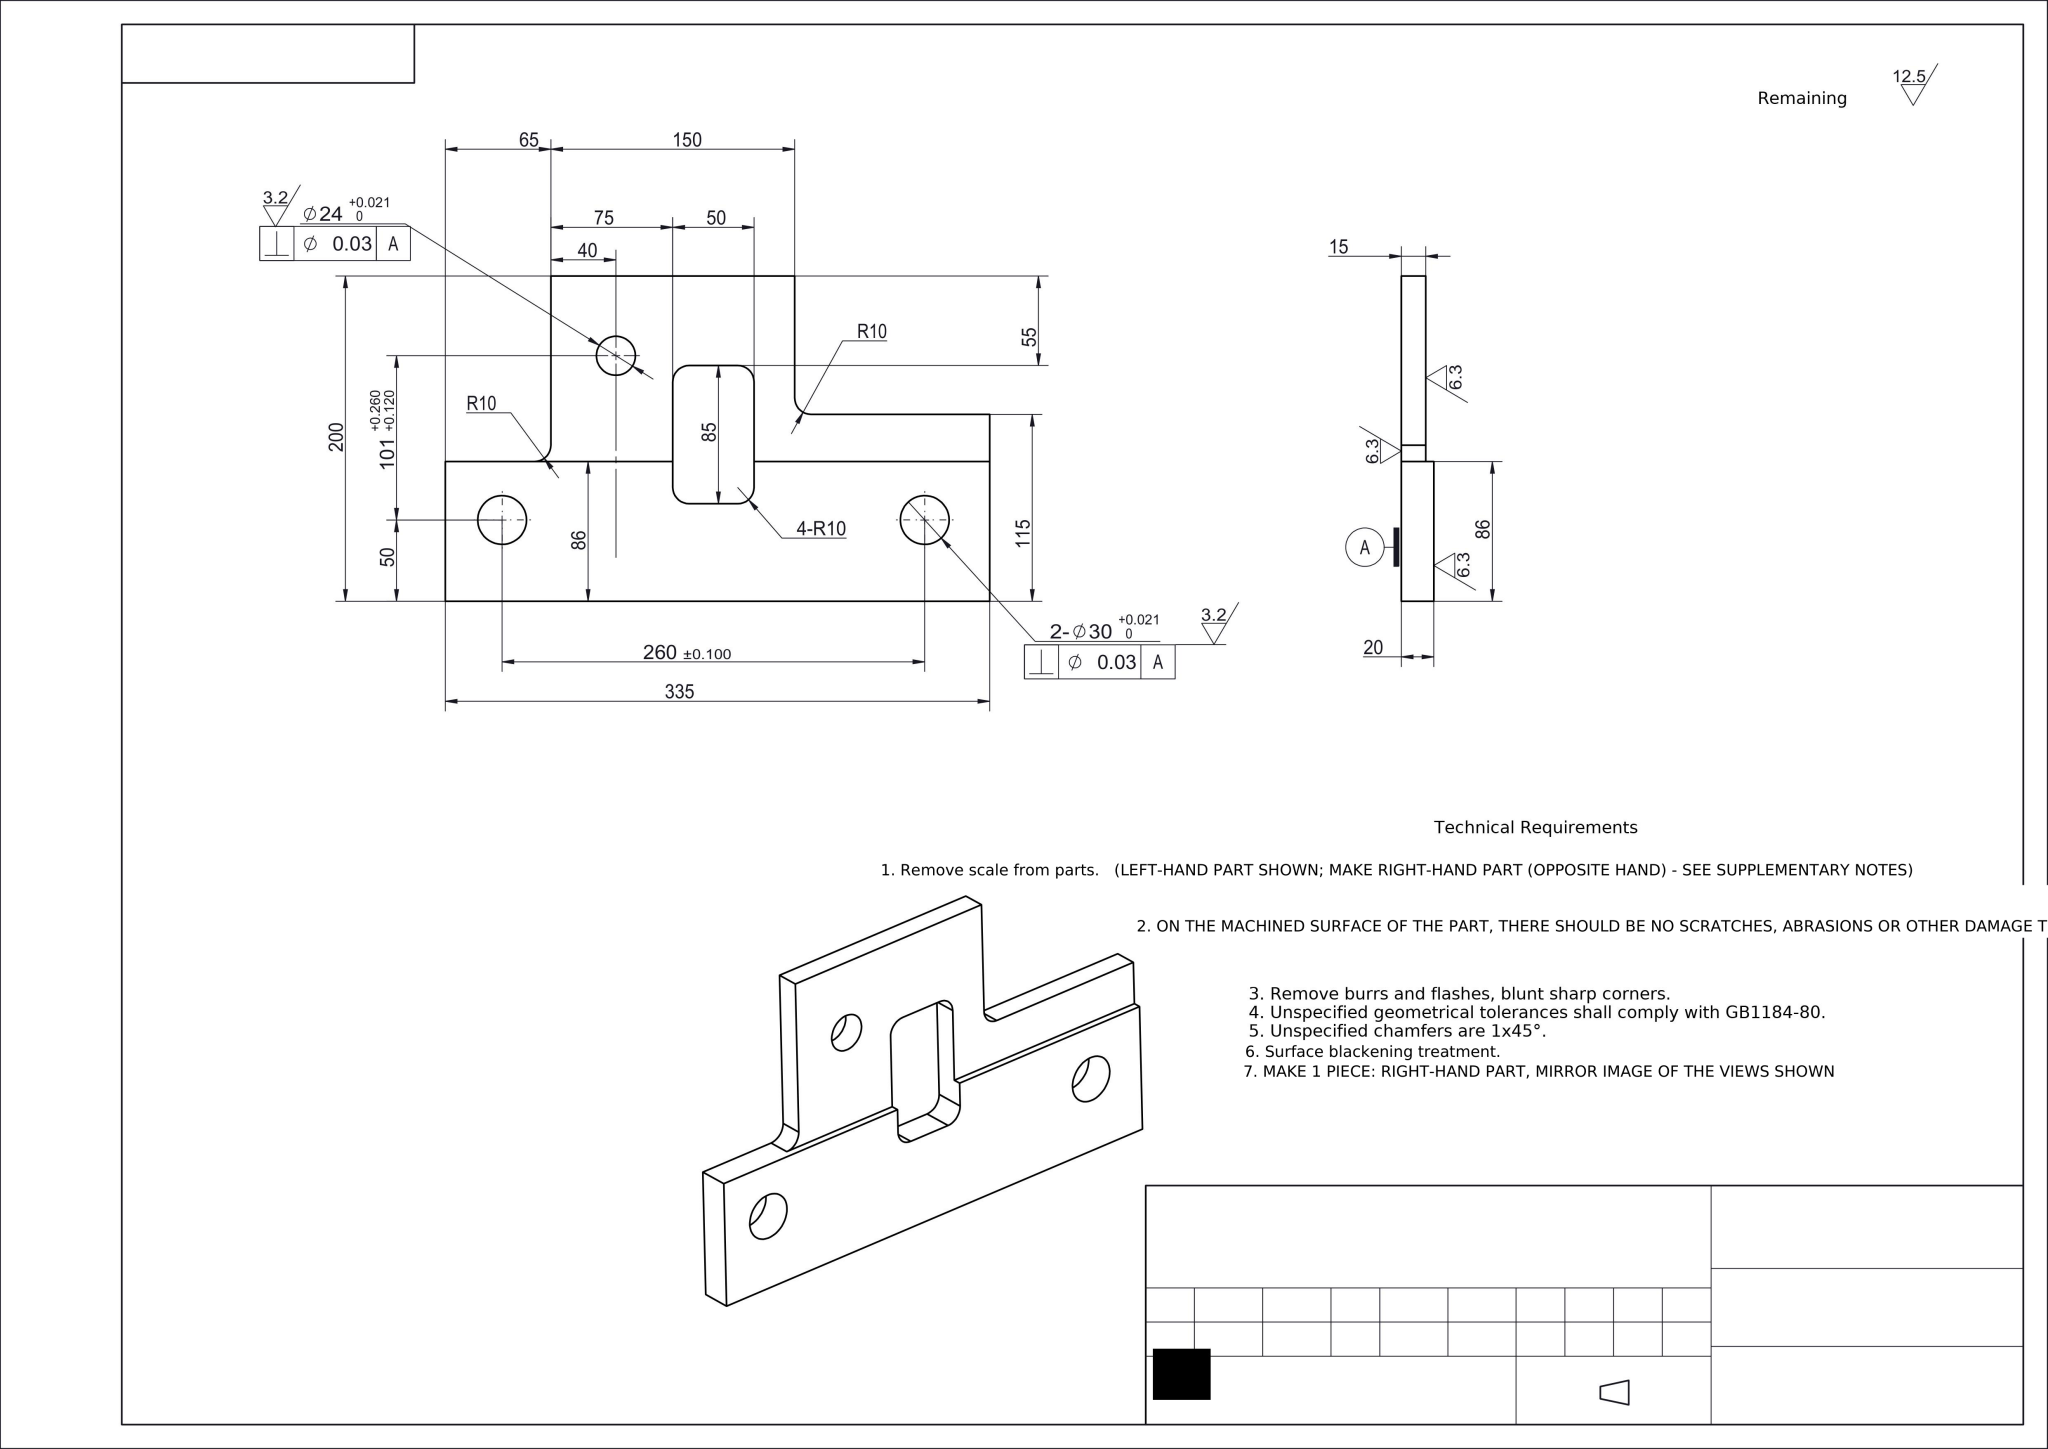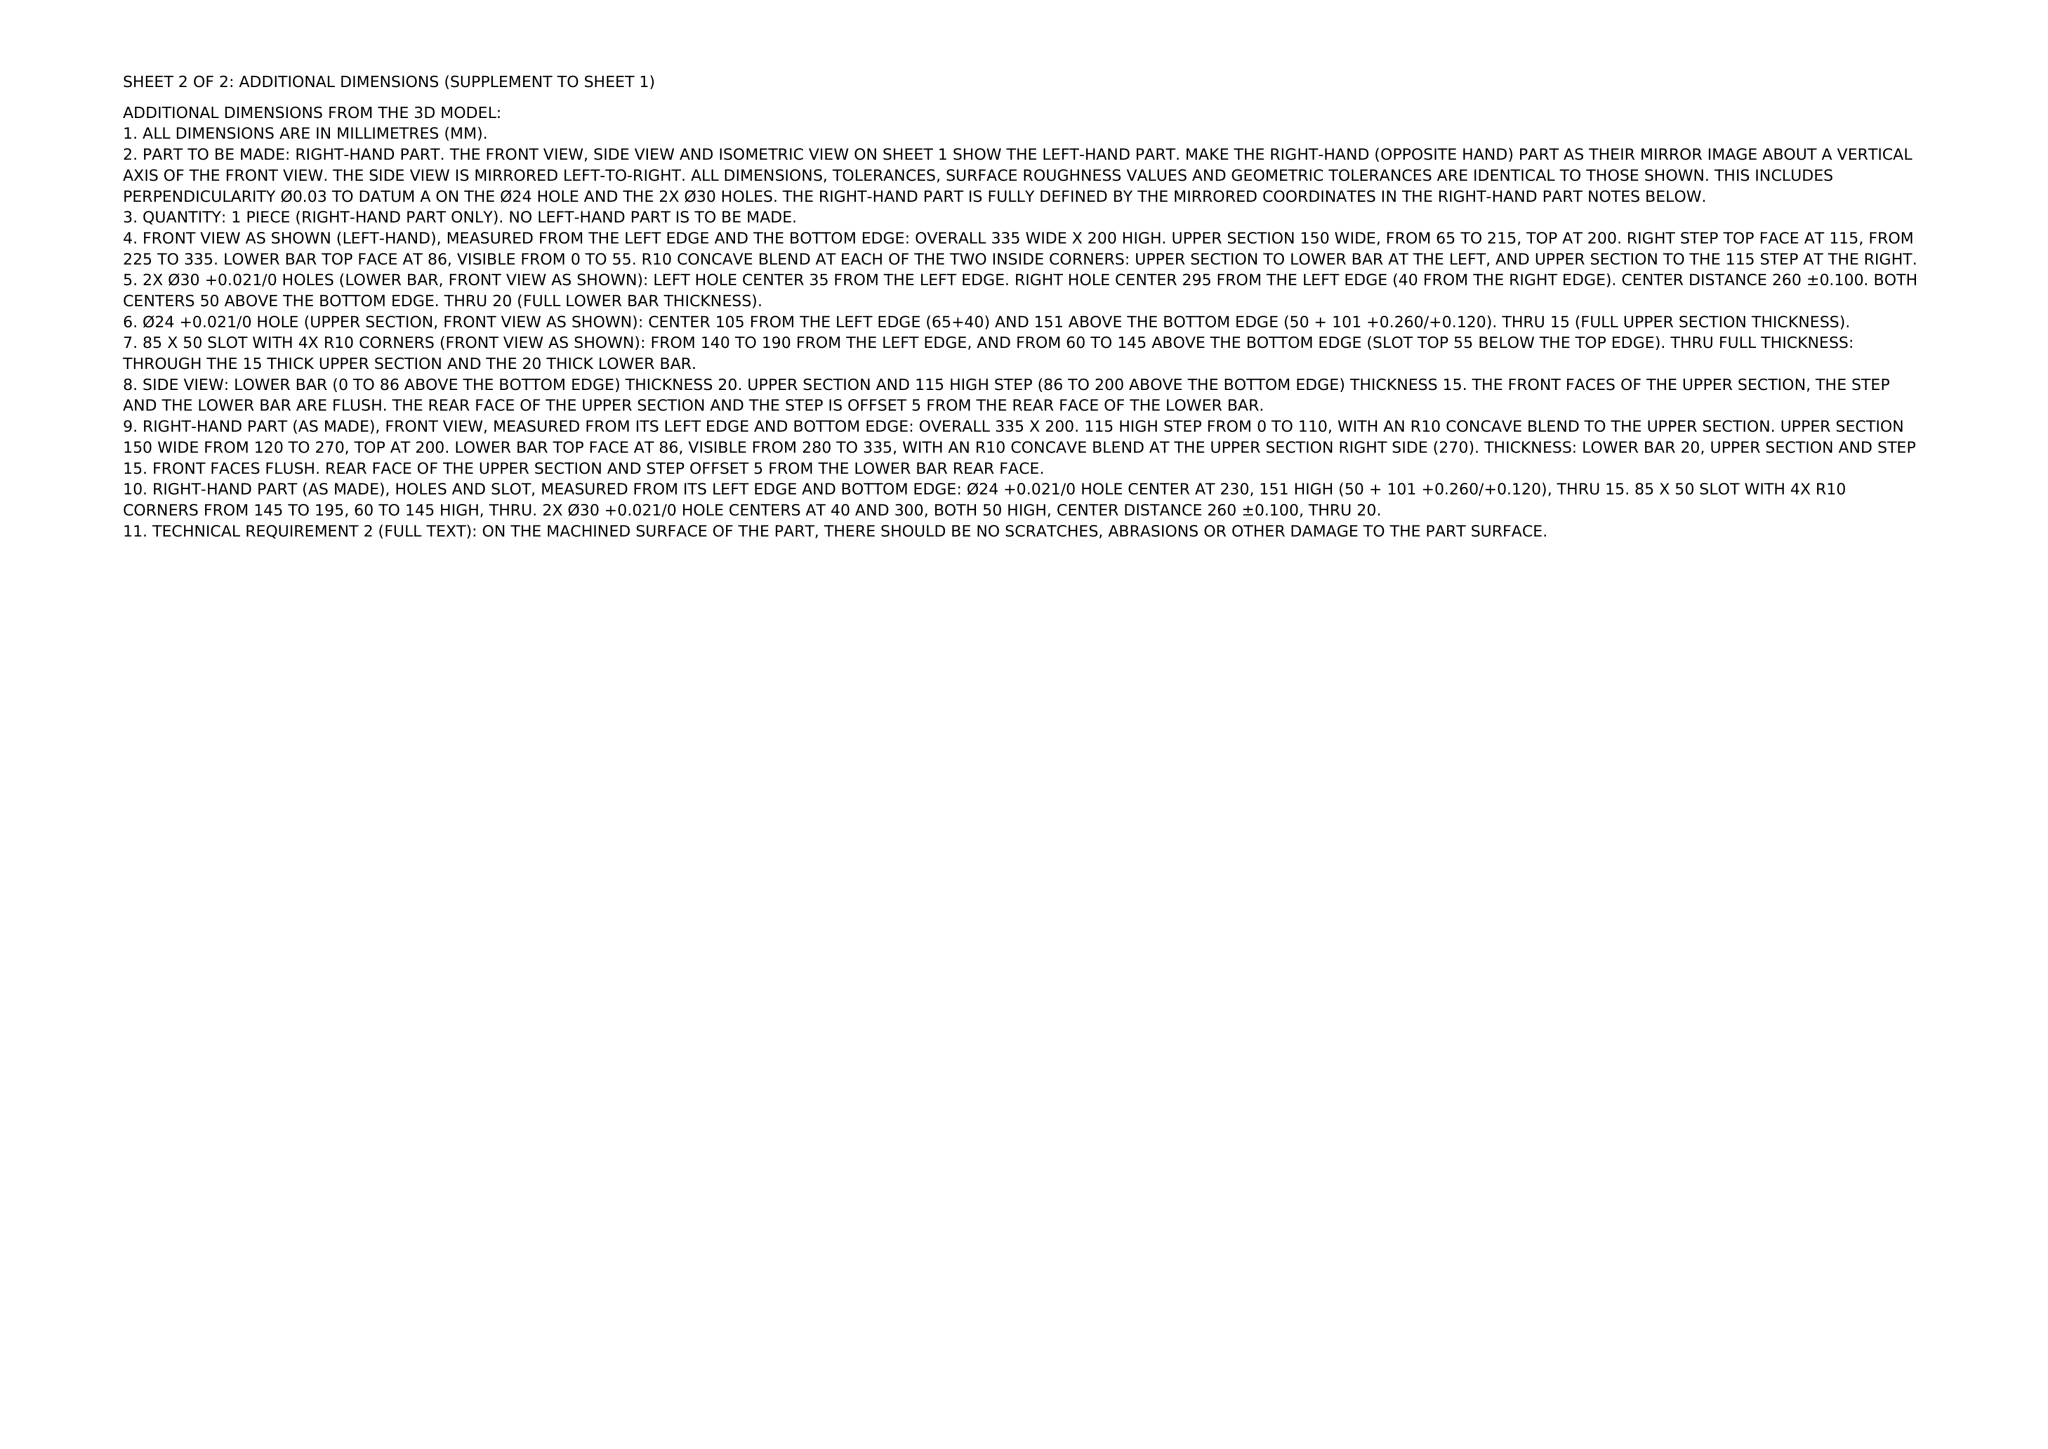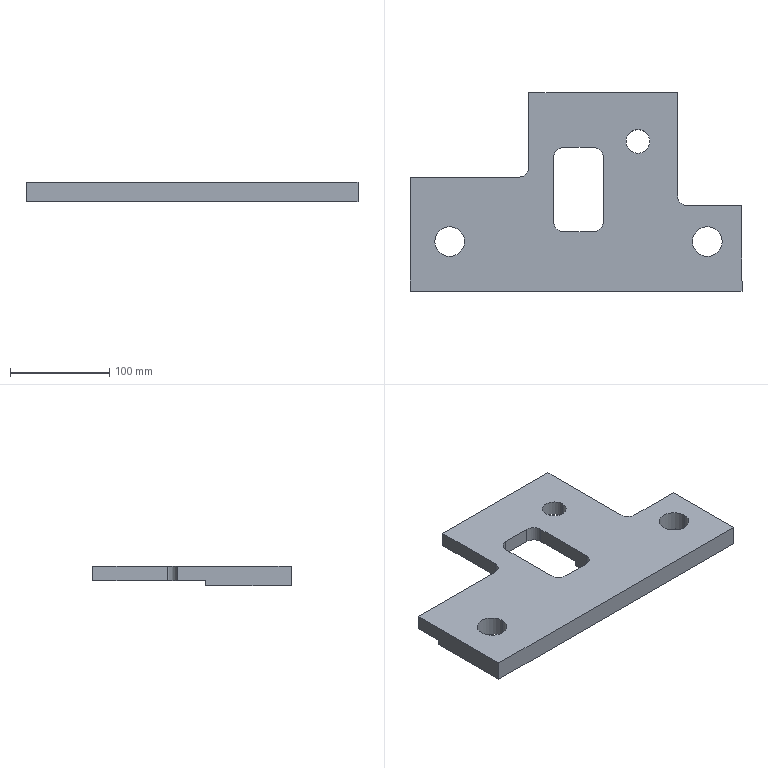Part | NX | mm | 1 solid | 28 faces | box 335 x 200 x 20 mm | volume 781736 mm3 | plane 16 | cylinder 12 | commonest cylinder face diameters 20 x6 30 x4 24 x2